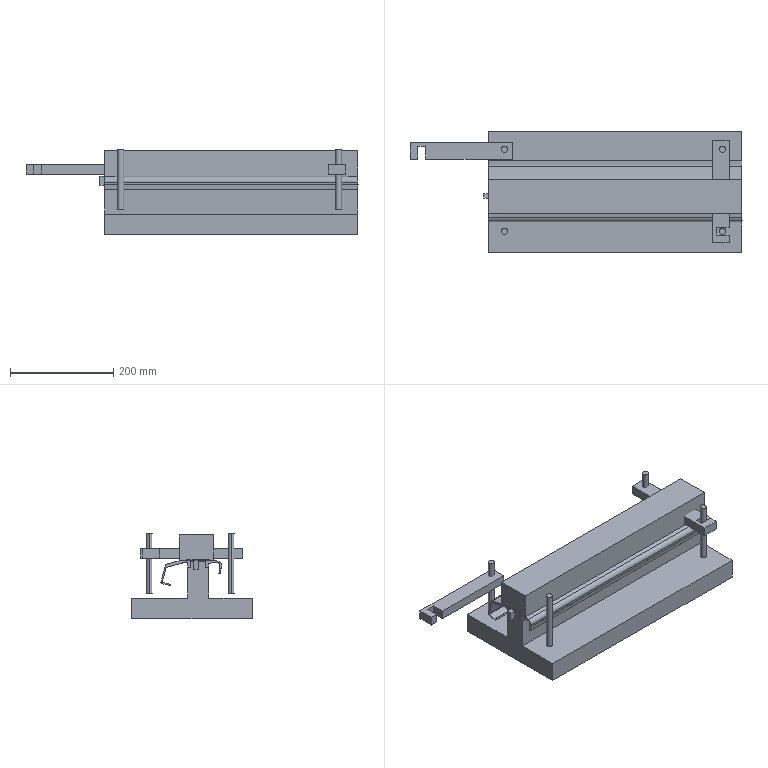CAM job | Mastercam | mm | 8 operations | part box 641.74 x 233.28 x 165.22
1. Contour (Ramp) | 1 - 16 平铣刀
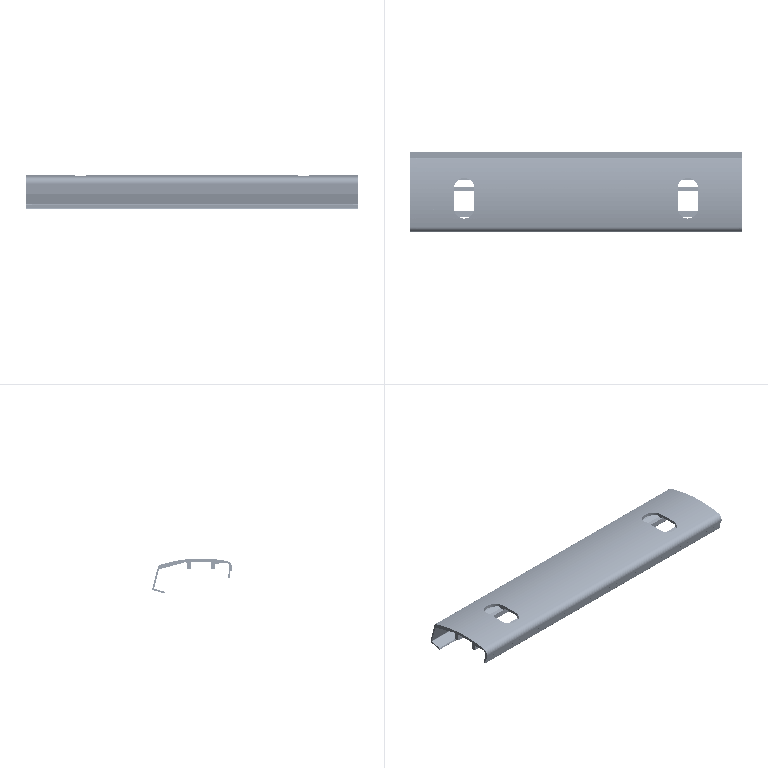2. Contour (Ramp) | 2 - 10 平铣刀
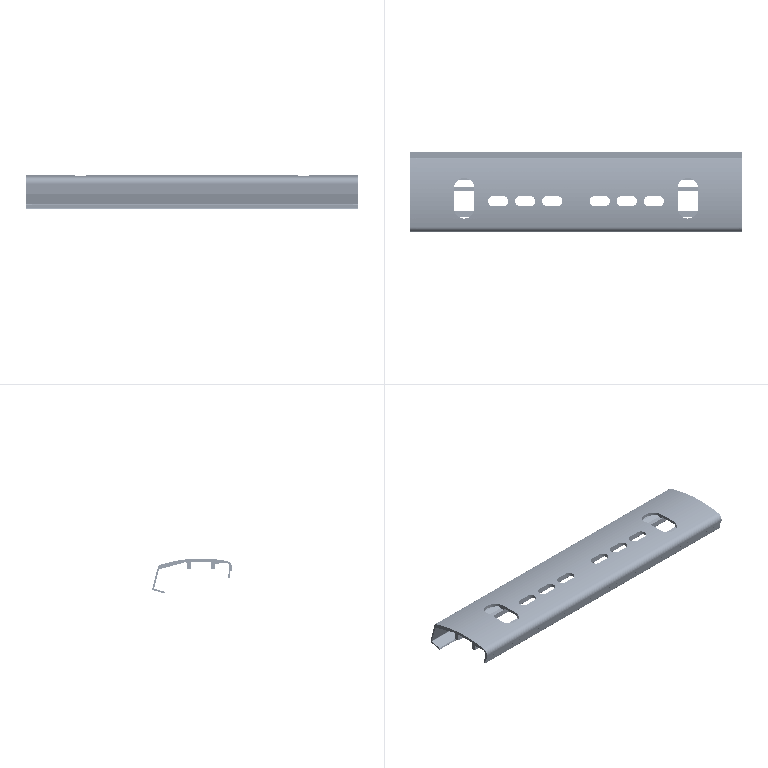3. Contour (2D) | 2 - 10 平铣刀
4. Contour (3D chamfer) | 3 - 5 倒角刀
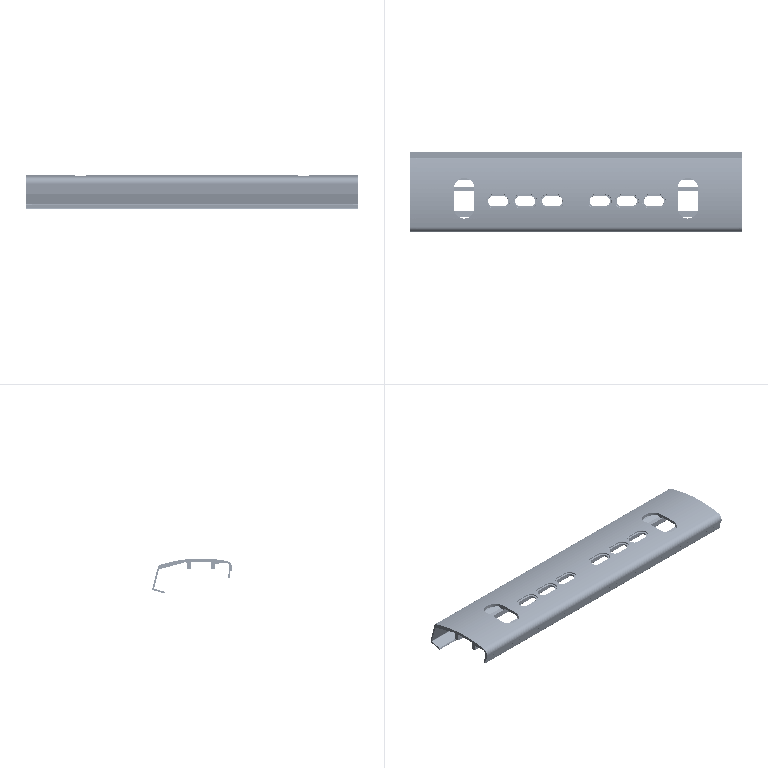5. Contour (3D chamfer) | 3 - 5 倒角刀
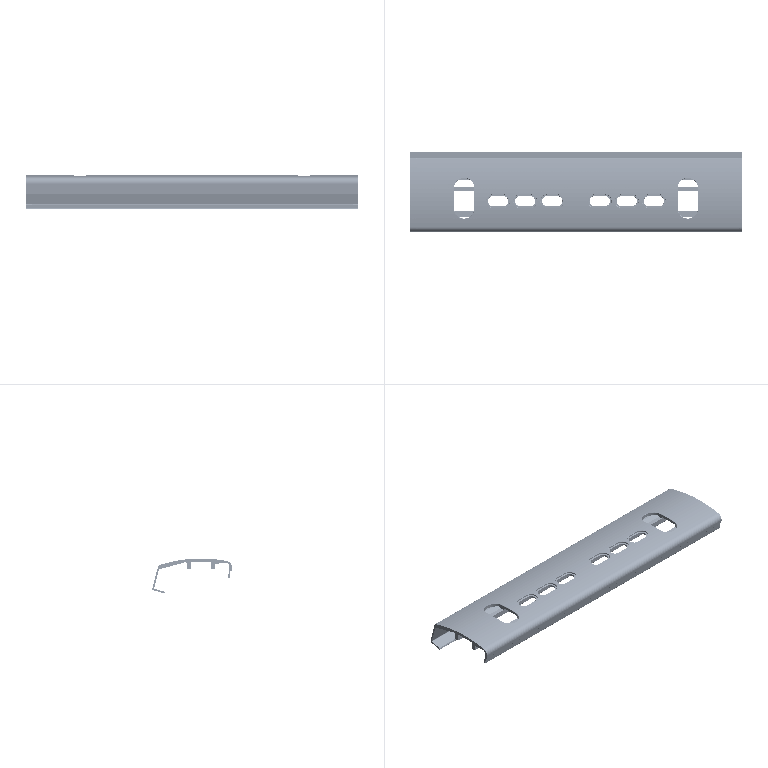6. Contour (2D) | 4 - 6 平铣刀
7. Contour (2D) | 4 - 6 平铣刀
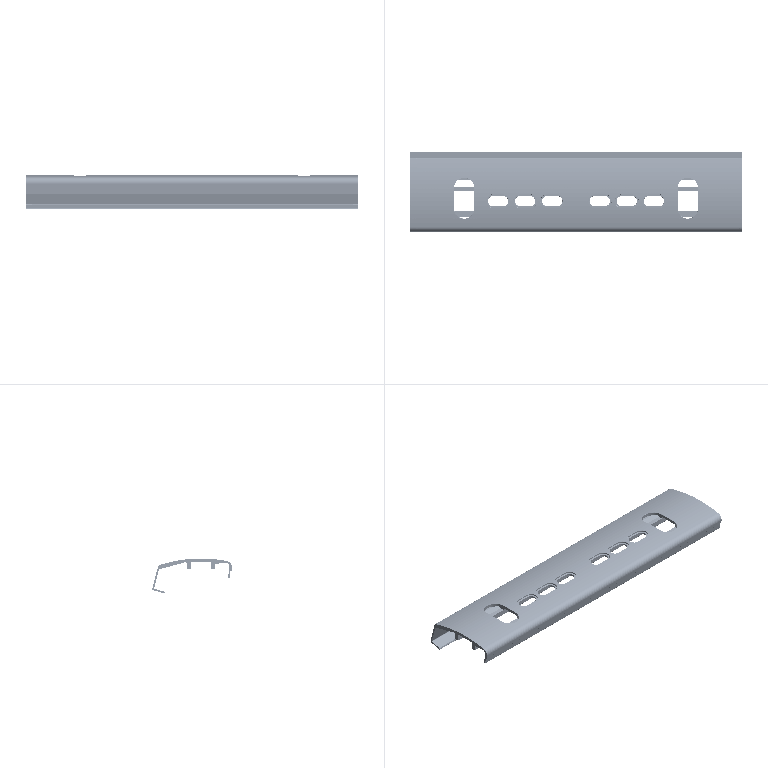8. Contour (2D) | 4 - 6 平铣刀